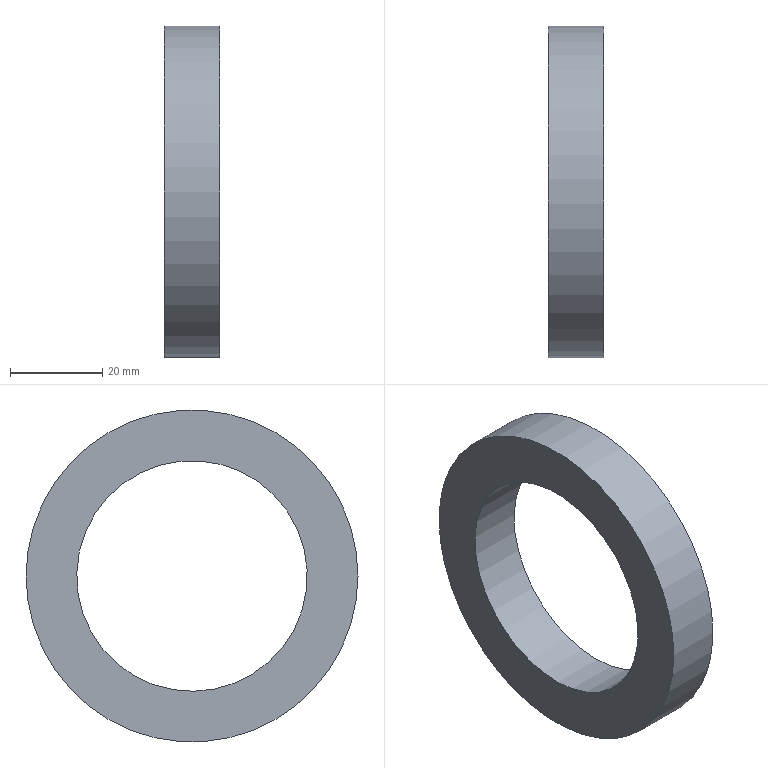Component | NX | OIL_SEAL_72X50X12 | 1 solid | 4 faces | box 12 x 72 x 72 mm | volume 25296 mm3 | cylinder 2 | plane 2 | commonest cylinder face diameters 72 x1 50 x1
STEP:
#1=CARTESIAN_POINT('',(0.,0.,0.));
#2=DIRECTION('',(0.,0.,1.));
#3=DIRECTION('',(1.,0.,0.));
#4=AXIS2_PLACEMENT_3D('',#1,#2,#3);
#5=CARTESIAN_POINT('',(307.,18.,-34.177));
#6=VERTEX_POINT('',#5);
#7=CARTESIAN_POINT('',(307.,0.,-3.));
#8=DIRECTION('',(1.,0.,0.));
#9=DIRECTION('',(0.,0.5,-0.866));
#10=AXIS2_PLACEMENT_3D('',#7,#8,#9);
#11=CIRCLE('',#10,36.);
#12=CARTESIAN_POINT('',(307.,0.,-3.));
#13=DIRECTION('',(-1.,0.,0.));
#14=DIRECTION('',(0.,-0.5,0.866));
#15=AXIS2_PLACEMENT_3D('',#12,#13,#14);
#16=CYLINDRICAL_SURFACE('',#15,36.);
#17=CARTESIAN_POINT('',(9.425,0.));
#18=DIRECTION('',(-1.,0.));
#19=VECTOR('',#18,1.);
#20=LINE('',#17,#19);
#21=(GEOMETRIC_REPRESENTATION_CONTEXT(2)PARAMETRIC_REPRESENTATION_CONTEXT()REPRESENTATION_CONTEXT('',''));
#22=DEFINITIONAL_REPRESENTATION('',(#20),#21);
#23=PCURVE('',#16,#22);
#24=CARTESIAN_POINT('',(307.,0.,-3.));
#25=DIRECTION('',(1.,0.,0.));
#26=DIRECTION('',(0.,0.5,-0.866));
#27=AXIS2_PLACEMENT_3D('',#24,#25,#26);
#28=PLANE('',#27);
#29=CARTESIAN_POINT('',(0.,0.));
#30=DIRECTION('',(1.,0.));
#31=AXIS2_PLACEMENT_2D('',#29,#30);
#32=CIRCLE('',#31,36.);
#33=(GEOMETRIC_REPRESENTATION_CONTEXT(2)PARAMETRIC_REPRESENTATION_CONTEXT()REPRESENTATION_CONTEXT('',''));
#34=DEFINITIONAL_REPRESENTATION('',(#32),#33);
#35=PCURVE('',#28,#34);
#36=SURFACE_CURVE('',#11,(#23,#35),.PCURVE_S1.);
#37=EDGE_CURVE('',#6,#6,#36,.T.);
#38=ORIENTED_EDGE('',*,*,#37,.F.);
#39=CARTESIAN_POINT('',(295.,18.,-34.177));
#40=VERTEX_POINT('',#39);
#41=CARTESIAN_POINT('',(307.,18.,-34.177));
#42=CARTESIAN_POINT('',(295.,18.,-34.177));
#43=B_SPLINE_CURVE_WITH_KNOTS('',1,(#41,#42),.UNSPECIFIED.,.F.,.F.,(2,2),(0.,12.),.PIECEWISE_BEZIER_KNOTS.);
#44=CARTESIAN_POINT('',(9.425,0.));
#45=DIRECTION('',(0.,1.));
#46=VECTOR('',#45,1.);
#47=LINE('',#44,#46);
#48=(GEOMETRIC_REPRESENTATION_CONTEXT(2)PARAMETRIC_REPRESENTATION_CONTEXT()REPRESENTATION_CONTEXT('',''));
#49=DEFINITIONAL_REPRESENTATION('',(#47),#48);
#50=PCURVE('',#16,#49);
#51=CARTESIAN_POINT('',(3.142,0.));
#52=DIRECTION('',(0.,1.));
#53=VECTOR('',#52,1.);
#54=LINE('',#51,#53);
#55=(GEOMETRIC_REPRESENTATION_CONTEXT(2)PARAMETRIC_REPRESENTATION_CONTEXT()REPRESENTATION_CONTEXT('',''));
#56=DEFINITIONAL_REPRESENTATION('',(#54),#55);
#57=PCURVE('',#16,#56);
#58=SEAM_CURVE('',#43,(#50,#57),.PCURVE_S1.);
#59=EDGE_CURVE('',#6,#40,#58,.T.);
#60=ORIENTED_EDGE('',*,*,#59,.T.);
#61=CARTESIAN_POINT('',(295.,0.,-3.));
#62=DIRECTION('',(1.,0.,0.));
#63=DIRECTION('',(0.,0.5,-0.866));
#64=AXIS2_PLACEMENT_3D('',#61,#62,#63);
#65=CIRCLE('',#64,36.);
#66=CARTESIAN_POINT('',(9.425,12.));
#67=DIRECTION('',(-1.,0.));
#68=VECTOR('',#67,1.);
#69=LINE('',#66,#68);
#70=(GEOMETRIC_REPRESENTATION_CONTEXT(2)PARAMETRIC_REPRESENTATION_CONTEXT()REPRESENTATION_CONTEXT('',''));
#71=DEFINITIONAL_REPRESENTATION('',(#69),#70);
#72=PCURVE('',#16,#71);
#73=CARTESIAN_POINT('',(295.,0.,-3.));
#74=DIRECTION('',(1.,0.,0.));
#75=DIRECTION('',(0.,0.5,-0.866));
#76=AXIS2_PLACEMENT_3D('',#73,#74,#75);
#77=PLANE('',#76);
#78=CARTESIAN_POINT('',(0.,0.));
#79=DIRECTION('',(1.,0.));
#80=AXIS2_PLACEMENT_2D('',#78,#79);
#81=CIRCLE('',#80,36.);
#82=(GEOMETRIC_REPRESENTATION_CONTEXT(2)PARAMETRIC_REPRESENTATION_CONTEXT()REPRESENTATION_CONTEXT('',''));
#83=DEFINITIONAL_REPRESENTATION('',(#81),#82);
#84=PCURVE('',#77,#83);
#85=SURFACE_CURVE('',#65,(#72,#84),.PCURVE_S1.);
#86=EDGE_CURVE('',#40,#40,#85,.T.);
#87=ORIENTED_EDGE('',*,*,#86,.T.);
#88=ORIENTED_EDGE('',*,*,#59,.F.);
#89=EDGE_LOOP('',(#38,#60,#87,#88));
#90=FACE_BOUND('',#89,.T.);
#91=ADVANCED_FACE('',(#90),#16,.T.);
#92=CARTESIAN_POINT('',(307.,12.5,-24.651));
#93=VERTEX_POINT('',#92);
#94=CARTESIAN_POINT('',(307.,0.,-3.));
#95=DIRECTION('',(1.,0.,0.));
#96=DIRECTION('',(0.,0.5,-0.866));
#97=AXIS2_PLACEMENT_3D('',#94,#95,#96);
#98=CIRCLE('',#97,25.);
#99=CARTESIAN_POINT('',(307.,0.,-3.));
#100=DIRECTION('',(-1.,0.,0.));
#101=DIRECTION('',(0.,-0.5,0.866));
#102=AXIS2_PLACEMENT_3D('',#99,#100,#101);
#103=CYLINDRICAL_SURFACE('',#102,25.);
#104=CARTESIAN_POINT('',(9.425,0.));
#105=DIRECTION('',(-1.,0.));
#106=VECTOR('',#105,1.);
#107=LINE('',#104,#106);
#108=(GEOMETRIC_REPRESENTATION_CONTEXT(2)PARAMETRIC_REPRESENTATION_CONTEXT()REPRESENTATION_CONTEXT('',''));
#109=DEFINITIONAL_REPRESENTATION('',(#107),#108);
#110=PCURVE('',#103,#109);
#111=CARTESIAN_POINT('',(0.,0.));
#112=DIRECTION('',(1.,0.));
#113=AXIS2_PLACEMENT_2D('',#111,#112);
#114=CIRCLE('',#113,25.);
#115=(GEOMETRIC_REPRESENTATION_CONTEXT(2)PARAMETRIC_REPRESENTATION_CONTEXT()REPRESENTATION_CONTEXT('',''));
#116=DEFINITIONAL_REPRESENTATION('',(#114),#115);
#117=PCURVE('',#28,#116);
#118=SURFACE_CURVE('',#98,(#110,#117),.PCURVE_S1.);
#119=EDGE_CURVE('',#93,#93,#118,.T.);
#120=ORIENTED_EDGE('',*,*,#119,.F.);
#121=CARTESIAN_POINT('',(295.,12.5,-24.651));
#122=VERTEX_POINT('',#121);
#123=CARTESIAN_POINT('',(307.,12.5,-24.651));
#124=CARTESIAN_POINT('',(295.,12.5,-24.651));
#125=B_SPLINE_CURVE_WITH_KNOTS('',1,(#123,#124),.UNSPECIFIED.,.F.,.F.,(2,2),(0.,12.),.PIECEWISE_BEZIER_KNOTS.);
#126=CARTESIAN_POINT('',(9.425,0.));
#127=DIRECTION('',(0.,1.));
#128=VECTOR('',#127,1.);
#129=LINE('',#126,#128);
#130=(GEOMETRIC_REPRESENTATION_CONTEXT(2)PARAMETRIC_REPRESENTATION_CONTEXT()REPRESENTATION_CONTEXT('',''));
#131=DEFINITIONAL_REPRESENTATION('',(#129),#130);
#132=PCURVE('',#103,#131);
#133=CARTESIAN_POINT('',(3.142,0.));
#134=DIRECTION('',(0.,1.));
#135=VECTOR('',#134,1.);
#136=LINE('',#133,#135);
#137=(GEOMETRIC_REPRESENTATION_CONTEXT(2)PARAMETRIC_REPRESENTATION_CONTEXT()REPRESENTATION_CONTEXT('',''));
#138=DEFINITIONAL_REPRESENTATION('',(#136),#137);
#139=PCURVE('',#103,#138);
#140=SEAM_CURVE('',#125,(#132,#139),.PCURVE_S1.);
#141=EDGE_CURVE('',#93,#122,#140,.T.);
#142=ORIENTED_EDGE('',*,*,#141,.T.);
#143=CARTESIAN_POINT('',(295.,0.,-3.));
#144=DIRECTION('',(1.,0.,0.));
#145=DIRECTION('',(0.,0.5,-0.866));
#146=AXIS2_PLACEMENT_3D('',#143,#144,#145);
#147=CIRCLE('',#146,25.);
#148=CARTESIAN_POINT('',(9.425,12.));
#149=DIRECTION('',(-1.,0.));
#150=VECTOR('',#149,1.);
#151=LINE('',#148,#150);
#152=(GEOMETRIC_REPRESENTATION_CONTEXT(2)PARAMETRIC_REPRESENTATION_CONTEXT()REPRESENTATION_CONTEXT('',''));
#153=DEFINITIONAL_REPRESENTATION('',(#151),#152);
#154=PCURVE('',#103,#153);
#155=CARTESIAN_POINT('',(0.,0.));
#156=DIRECTION('',(1.,0.));
#157=AXIS2_PLACEMENT_2D('',#155,#156);
#158=CIRCLE('',#157,25.);
#159=(GEOMETRIC_REPRESENTATION_CONTEXT(2)PARAMETRIC_REPRESENTATION_CONTEXT()REPRESENTATION_CONTEXT('',''));
#160=DEFINITIONAL_REPRESENTATION('',(#158),#159);
#161=PCURVE('',#77,#160);
#162=SURFACE_CURVE('',#147,(#154,#161),.PCURVE_S1.);
#163=EDGE_CURVE('',#122,#122,#162,.T.);
#164=ORIENTED_EDGE('',*,*,#163,.T.);
#165=ORIENTED_EDGE('',*,*,#141,.F.);
#166=EDGE_LOOP('',(#120,#142,#164,#165));
#167=FACE_BOUND('',#166,.F.);
#168=ADVANCED_FACE('',(#167),#103,.F.);
#169=ORIENTED_EDGE('',*,*,#37,.T.);
#170=EDGE_LOOP('',(#169));
#171=FACE_BOUND('',#170,.T.);
#172=ORIENTED_EDGE('',*,*,#119,.F.);
#173=EDGE_LOOP('',(#172));
#174=FACE_BOUND('',#173,.T.);
#175=ADVANCED_FACE('',(#171,#174),#28,.T.);
#176=ORIENTED_EDGE('',*,*,#86,.F.);
#177=EDGE_LOOP('',(#176));
#178=FACE_BOUND('',#177,.T.);
#179=ORIENTED_EDGE('',*,*,#163,.T.);
#180=EDGE_LOOP('',(#179));
#181=FACE_BOUND('',#180,.T.);
#182=ADVANCED_FACE('',(#178,#181),#77,.F.);
#183=CLOSED_SHELL('',(#91,#168,#175,#182));
#184=MANIFOLD_SOLID_BREP('',#183);
#185=(LENGTH_UNIT()NAMED_UNIT(*)SI_UNIT(.MILLI.,.METRE.));
#186=UNCERTAINTY_MEASURE_WITH_UNIT(LENGTH_MEASURE(0.00001),#185,'','');
#187=(NAMED_UNIT(*)PLANE_ANGLE_UNIT()SI_UNIT($,.RADIAN.));
#188=(NAMED_UNIT(*)SI_UNIT($,.STERADIAN.)SOLID_ANGLE_UNIT());
#189=(GEOMETRIC_REPRESENTATION_CONTEXT(3)GLOBAL_UNCERTAINTY_ASSIGNED_CONTEXT((#186))GLOBAL_UNIT_ASSIGNED_CONTEXT((#185,#187,#188))REPRESENTATION_CONTEXT('',''));
#190=ADVANCED_BREP_SHAPE_REPRESENTATION('',(#4,#184),#189);